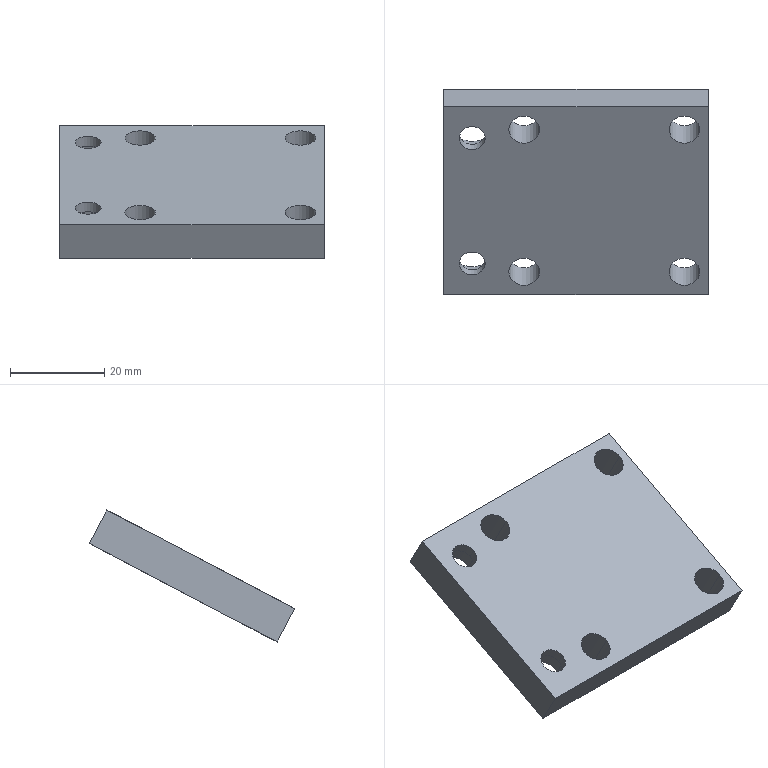Component | SolidWorks | SDACylinderFixingPlate-1 | 1 solid | 24 faces | box 56 x 43.56 x 28 mm | volume 18093 mm3 | cylinder 16 | plane 8 | commonest cylinder face diameters 6.5 x8 10 x4 5.5 x4
build123d program:
from build123d import *

# Parameters (mm, degrees)
SKETCH1_W                                          = 56
SKETCH1_H                                          = 45
BOSS_EXTRUDE1_DEPTH                                = 8
HOLE_SIZE_ACCORDING_TO_TYPE_1_OF_HEXAG_D           = 5.5
HOLE_SIZE_ACCORDING_TO_TYPE_1_OF_HEXAG_CBORE_D     = 10
HOLE_SIZE_ACCORDING_TO_TYPE_1_OF_HEXAG_CBORE_DEPTH = 5.7
F_6_5_6_5_DIAMETER_HOLE1_D                         = 6.5


with BuildPart() as part:
    # Sketch1 → Boss-Extrude1 (new body)
    with BuildSketch(Plane.XY):
        Rectangle(SKETCH1_W, SKETCH1_H)
    extrude(amount=BOSS_EXTRUDE1_DEPTH)

    # Hole Size _according to_ Type 1 of Hexag (through all)
    with Locations(Plane.XY.offset(8)):
        with Locations((22, 15), (22, -15)):
            CounterBoreHole(HOLE_SIZE_ACCORDING_TO_TYPE_1_OF_HEXAG_D / 2, HOLE_SIZE_ACCORDING_TO_TYPE_1_OF_HEXAG_CBORE_D / 2, HOLE_SIZE_ACCORDING_TO_TYPE_1_OF_HEXAG_CBORE_DEPTH)

    # 6.5 _6.5_ Diameter Hole1 (through all)
    with Locations(Plane.XY.offset(8)):
        with Locations((-23, 17), (11, 17), (11, -17), (-23, -17)):
            Hole(F_6_5_6_5_DIAMETER_HOLE1_D / 2)


solid = part.part

# Placed as in the assembly
solid = solid.moved(Location((-251.317, 16.632, 98.15), (-152.302, 0, 180)))
STEP:
#1=CARTESIAN_POINT('',(-8.861,1.247,4.175));
#2=VERTEX_POINT('',#1);
#3=CARTESIAN_POINT('',(-9.117,1.247,4.175));
#4=VERTEX_POINT('',#3);
#5=CARTESIAN_POINT('',(-8.989,1.247,4.175));
#6=DIRECTION('',(-0.,0.4648,-0.8854));
#7=DIRECTION('',(-1.,-0.,0.));
#8=AXIS2_PLACEMENT_3D('',#5,#6,#7);
#9=CIRCLE('',#8,0.128);
#10=EDGE_CURVE('',#2,#4,#9,.T.);
#11=ORIENTED_EDGE('',*,*,#10,.F.);
#12=CARTESIAN_POINT('',(-8.861,1.394,3.896));
#13=VERTEX_POINT('',#12);
#14=CARTESIAN_POINT('',(-8.861,1.394,3.896));
#15=DIRECTION('',(-0.,0.4648,-0.8854));
#16=VECTOR('',#15,39.37);
#17=LINE('',#14,#16);
#18=EDGE_CURVE('',#2,#13,#17,.T.);
#19=ORIENTED_EDGE('',*,*,#18,.T.);
#20=CARTESIAN_POINT('',(-9.117,1.394,3.896));
#21=VERTEX_POINT('',#20);
#22=CARTESIAN_POINT('',(-8.989,1.394,3.896));
#23=DIRECTION('',(-0.,0.4648,-0.8854));
#24=DIRECTION('',(-1.,-0.,0.));
#25=AXIS2_PLACEMENT_3D('',#22,#23,#24);
#26=CIRCLE('',#25,0.128);
#27=EDGE_CURVE('',#13,#21,#26,.T.);
#28=ORIENTED_EDGE('',*,*,#27,.T.);
#29=CARTESIAN_POINT('',(-9.117,1.394,3.896));
#30=DIRECTION('',(-0.,0.4648,-0.8854));
#31=VECTOR('',#30,39.37);
#32=LINE('',#29,#31);
#33=EDGE_CURVE('',#4,#21,#32,.T.);
#34=ORIENTED_EDGE('',*,*,#33,.F.);
#35=EDGE_LOOP('',(#11,#19,#28,#34));
#36=FACE_OUTER_BOUND('',#35,.T.);
#37=CARTESIAN_POINT('',(-8.989,1.394,3.896));
#38=DIRECTION('',(-0.,0.4648,-0.8854));
#39=DIRECTION('',(-1.,-0.,0.));
#40=AXIS2_PLACEMENT_3D('',#37,#38,#39);
#41=CYLINDRICAL_SURFACE('',#40,0.128);
#42=ADVANCED_FACE('',(#36),#41,.F.);
#43=CARTESIAN_POINT('',(-10.199,1.247,4.175));
#44=VERTEX_POINT('',#43);
#45=CARTESIAN_POINT('',(-10.455,1.247,4.175));
#46=VERTEX_POINT('',#45);
#47=CARTESIAN_POINT('',(-10.327,1.247,4.175));
#48=DIRECTION('',(-0.,0.4648,-0.8854));
#49=DIRECTION('',(-1.,-0.,0.));
#50=AXIS2_PLACEMENT_3D('',#47,#48,#49);
#51=CIRCLE('',#50,0.128);
#52=EDGE_CURVE('',#44,#46,#51,.T.);
#53=ORIENTED_EDGE('',*,*,#52,.F.);
#54=CARTESIAN_POINT('',(-10.199,1.394,3.896));
#55=VERTEX_POINT('',#54);
#56=CARTESIAN_POINT('',(-10.199,1.394,3.896));
#57=DIRECTION('',(-0.,0.4648,-0.8854));
#58=VECTOR('',#57,39.37);
#59=LINE('',#56,#58);
#60=EDGE_CURVE('',#44,#55,#59,.T.);
#61=ORIENTED_EDGE('',*,*,#60,.T.);
#62=CARTESIAN_POINT('',(-10.455,1.394,3.896));
#63=VERTEX_POINT('',#62);
#64=CARTESIAN_POINT('',(-10.327,1.394,3.896));
#65=DIRECTION('',(-0.,0.4648,-0.8854));
#66=DIRECTION('',(-1.,-0.,0.));
#67=AXIS2_PLACEMENT_3D('',#64,#65,#66);
#68=CIRCLE('',#67,0.128);
#69=EDGE_CURVE('',#55,#63,#68,.T.);
#70=ORIENTED_EDGE('',*,*,#69,.T.);
#71=CARTESIAN_POINT('',(-10.455,1.394,3.896));
#72=DIRECTION('',(-0.,0.4648,-0.8854));
#73=VECTOR('',#72,39.37);
#74=LINE('',#71,#73);
#75=EDGE_CURVE('',#46,#63,#74,.T.);
#76=ORIENTED_EDGE('',*,*,#75,.F.);
#77=EDGE_LOOP('',(#53,#61,#70,#76));
#78=FACE_OUTER_BOUND('',#77,.T.);
#79=CARTESIAN_POINT('',(-10.327,1.394,3.896));
#80=DIRECTION('',(-0.,0.4648,-0.8854));
#81=DIRECTION('',(-1.,-0.,0.));
#82=AXIS2_PLACEMENT_3D('',#79,#80,#81);
#83=CYLINDRICAL_SURFACE('',#82,0.128);
#84=ADVANCED_FACE('',(#78),#83,.F.);
#85=CARTESIAN_POINT('',(-10.199,0.06221,3.553));
#86=VERTEX_POINT('',#85);
#87=CARTESIAN_POINT('',(-10.455,0.06221,3.553));
#88=VERTEX_POINT('',#87);
#89=CARTESIAN_POINT('',(-10.327,0.06221,3.553));
#90=DIRECTION('',(-0.,0.4648,-0.8854));
#91=DIRECTION('',(-1.,-0.,0.));
#92=AXIS2_PLACEMENT_3D('',#89,#90,#91);
#93=CIRCLE('',#92,0.128);
#94=EDGE_CURVE('',#86,#88,#93,.T.);
#95=ORIENTED_EDGE('',*,*,#94,.F.);
#96=CARTESIAN_POINT('',(-10.199,0.2086,3.274));
#97=VERTEX_POINT('',#96);
#98=CARTESIAN_POINT('',(-10.199,0.2086,3.274));
#99=DIRECTION('',(-0.,0.4648,-0.8854));
#100=VECTOR('',#99,39.37);
#101=LINE('',#98,#100);
#102=EDGE_CURVE('',#86,#97,#101,.T.);
#103=ORIENTED_EDGE('',*,*,#102,.T.);
#104=CARTESIAN_POINT('',(-10.455,0.2086,3.274));
#105=VERTEX_POINT('',#104);
#106=CARTESIAN_POINT('',(-10.327,0.2086,3.274));
#107=DIRECTION('',(-0.,0.4648,-0.8854));
#108=DIRECTION('',(-1.,-0.,0.));
#109=AXIS2_PLACEMENT_3D('',#106,#107,#108);
#110=CIRCLE('',#109,0.128);
#111=EDGE_CURVE('',#97,#105,#110,.T.);
#112=ORIENTED_EDGE('',*,*,#111,.T.);
#113=CARTESIAN_POINT('',(-10.455,0.2086,3.274));
#114=DIRECTION('',(-0.,0.4648,-0.8854));
#115=VECTOR('',#114,39.37);
#116=LINE('',#113,#115);
#117=EDGE_CURVE('',#88,#105,#116,.T.);
#118=ORIENTED_EDGE('',*,*,#117,.F.);
#119=EDGE_LOOP('',(#95,#103,#112,#118));
#120=FACE_OUTER_BOUND('',#119,.T.);
#121=CARTESIAN_POINT('',(-10.327,0.2086,3.274));
#122=DIRECTION('',(-0.,0.4648,-0.8854));
#123=DIRECTION('',(-1.,-0.,0.));
#124=AXIS2_PLACEMENT_3D('',#121,#122,#123);
#125=CYLINDRICAL_SURFACE('',#124,0.128);
#126=ADVANCED_FACE('',(#120),#125,.F.);
#127=CARTESIAN_POINT('',(-8.861,0.06221,3.553));
#128=VERTEX_POINT('',#127);
#129=CARTESIAN_POINT('',(-9.117,0.06221,3.553));
#130=VERTEX_POINT('',#129);
#131=CARTESIAN_POINT('',(-8.989,0.06221,3.553));
#132=DIRECTION('',(-0.,0.4648,-0.8854));
#133=DIRECTION('',(-1.,-0.,0.));
#134=AXIS2_PLACEMENT_3D('',#131,#132,#133);
#135=CIRCLE('',#134,0.128);
#136=EDGE_CURVE('',#128,#130,#135,.T.);
#137=ORIENTED_EDGE('',*,*,#136,.F.);
#138=CARTESIAN_POINT('',(-8.861,0.2086,3.274));
#139=VERTEX_POINT('',#138);
#140=CARTESIAN_POINT('',(-8.861,0.2086,3.274));
#141=DIRECTION('',(-0.,0.4648,-0.8854));
#142=VECTOR('',#141,39.37);
#143=LINE('',#140,#142);
#144=EDGE_CURVE('',#128,#139,#143,.T.);
#145=ORIENTED_EDGE('',*,*,#144,.T.);
#146=CARTESIAN_POINT('',(-9.117,0.2086,3.274));
#147=VERTEX_POINT('',#146);
#148=CARTESIAN_POINT('',(-8.989,0.2086,3.274));
#149=DIRECTION('',(-0.,0.4648,-0.8854));
#150=DIRECTION('',(-1.,-0.,0.));
#151=AXIS2_PLACEMENT_3D('',#148,#149,#150);
#152=CIRCLE('',#151,0.128);
#153=EDGE_CURVE('',#139,#147,#152,.T.);
#154=ORIENTED_EDGE('',*,*,#153,.T.);
#155=CARTESIAN_POINT('',(-9.117,0.2086,3.274));
#156=DIRECTION('',(-0.,0.4648,-0.8854));
#157=VECTOR('',#156,39.37);
#158=LINE('',#155,#157);
#159=EDGE_CURVE('',#130,#147,#158,.T.);
#160=ORIENTED_EDGE('',*,*,#159,.F.);
#161=EDGE_LOOP('',(#137,#145,#154,#160));
#162=FACE_OUTER_BOUND('',#161,.T.);
#163=CARTESIAN_POINT('',(-8.989,0.2086,3.274));
#164=DIRECTION('',(-0.,0.4648,-0.8854));
#165=DIRECTION('',(-1.,-0.,0.));
#166=AXIS2_PLACEMENT_3D('',#163,#164,#165);
#167=CYLINDRICAL_SURFACE('',#166,0.128);
#168=ADVANCED_FACE('',(#162),#167,.F.);
#169=CARTESIAN_POINT('',(-10.564,1.22,4.058));
#170=VERTEX_POINT('',#169);
#171=CARTESIAN_POINT('',(-10.957,1.22,4.058));
#172=VERTEX_POINT('',#171);
#173=CARTESIAN_POINT('',(-10.76,1.22,4.058));
#174=DIRECTION('',(-0.,0.4648,-0.8854));
#175=DIRECTION('',(-1.,-0.,0.));
#176=AXIS2_PLACEMENT_3D('',#173,#174,#175);
#177=CIRCLE('',#176,0.1969);
#178=EDGE_CURVE('',#170,#172,#177,.T.);
#179=ORIENTED_EDGE('',*,*,#178,.F.);
#180=CARTESIAN_POINT('',(-10.564,1.324,3.86));
#181=VERTEX_POINT('',#180);
#182=CARTESIAN_POINT('',(-10.564,1.324,3.86));
#183=DIRECTION('',(-0.,0.4648,-0.8854));
#184=VECTOR('',#183,39.37);
#185=LINE('',#182,#184);
#186=EDGE_CURVE('',#170,#181,#185,.T.);
#187=ORIENTED_EDGE('',*,*,#186,.T.);
#188=CARTESIAN_POINT('',(-10.957,1.324,3.86));
#189=VERTEX_POINT('',#188);
#190=CARTESIAN_POINT('',(-10.76,1.324,3.86));
#191=DIRECTION('',(-0.,0.4648,-0.8854));
#192=DIRECTION('',(-1.,-0.,0.));
#193=AXIS2_PLACEMENT_3D('',#190,#191,#192);
#194=CIRCLE('',#193,0.1969);
#195=EDGE_CURVE('',#181,#189,#194,.T.);
#196=ORIENTED_EDGE('',*,*,#195,.T.);
#197=CARTESIAN_POINT('',(-10.957,1.324,3.86));
#198=DIRECTION('',(-0.,0.4648,-0.8854));
#199=VECTOR('',#198,39.37);
#200=LINE('',#197,#199);
#201=EDGE_CURVE('',#172,#189,#200,.T.);
#202=ORIENTED_EDGE('',*,*,#201,.F.);
#203=EDGE_LOOP('',(#179,#187,#196,#202));
#204=FACE_OUTER_BOUND('',#203,.T.);
#205=CARTESIAN_POINT('',(-10.76,1.324,3.86));
#206=DIRECTION('',(-0.,0.4648,-0.8854));
#207=DIRECTION('',(-1.,-0.,0.));
#208=AXIS2_PLACEMENT_3D('',#205,#206,#207);
#209=CYLINDRICAL_SURFACE('',#208,0.1969);
#210=ADVANCED_FACE('',(#204),#209,.F.);
#211=CARTESIAN_POINT('',(-10.652,1.178,4.139));
#212=VERTEX_POINT('',#211);
#213=CARTESIAN_POINT('',(-10.869,1.178,4.139));
#214=VERTEX_POINT('',#213);
#215=CARTESIAN_POINT('',(-10.76,1.178,4.139));
#216=DIRECTION('',(-0.,0.4648,-0.8854));
#217=DIRECTION('',(-1.,-0.,0.));
#218=AXIS2_PLACEMENT_3D('',#215,#216,#217);
#219=CIRCLE('',#218,0.1083);
#220=EDGE_CURVE('',#212,#214,#219,.T.);
#221=ORIENTED_EDGE('',*,*,#220,.F.);
#222=CARTESIAN_POINT('',(-10.652,1.22,4.058));
#223=VERTEX_POINT('',#222);
#224=CARTESIAN_POINT('',(-10.652,1.324,3.86));
#225=DIRECTION('',(-0.,0.4648,-0.8854));
#226=VECTOR('',#225,39.37);
#227=LINE('',#224,#226);
#228=EDGE_CURVE('',#212,#223,#227,.T.);
#229=ORIENTED_EDGE('',*,*,#228,.T.);
#230=CARTESIAN_POINT('',(-10.869,1.22,4.058));
#231=VERTEX_POINT('',#230);
#232=CARTESIAN_POINT('',(-10.76,1.22,4.058));
#233=DIRECTION('',(-0.,0.4648,-0.8854));
#234=DIRECTION('',(-1.,-0.,0.));
#235=AXIS2_PLACEMENT_3D('',#232,#233,#234);
#236=CIRCLE('',#235,0.1083);
#237=EDGE_CURVE('',#223,#231,#236,.T.);
#238=ORIENTED_EDGE('',*,*,#237,.T.);
#239=CARTESIAN_POINT('',(-10.869,1.324,3.86));
#240=DIRECTION('',(-0.,0.4648,-0.8854));
#241=VECTOR('',#240,39.37);
#242=LINE('',#239,#241);
#243=EDGE_CURVE('',#214,#231,#242,.T.);
#244=ORIENTED_EDGE('',*,*,#243,.F.);
#245=EDGE_LOOP('',(#221,#229,#238,#244));
#246=FACE_OUTER_BOUND('',#245,.T.);
#247=CARTESIAN_POINT('',(-10.76,1.324,3.86));
#248=DIRECTION('',(-0.,0.4648,-0.8854));
#249=DIRECTION('',(-1.,-0.,0.));
#250=AXIS2_PLACEMENT_3D('',#247,#248,#249);
#251=CYLINDRICAL_SURFACE('',#250,0.1083);
#252=ADVANCED_FACE('',(#246),#251,.F.);
#253=CARTESIAN_POINT('',(-10.564,0.174,3.509));
#254=VERTEX_POINT('',#253);
#255=CARTESIAN_POINT('',(-10.957,0.174,3.509));
#256=VERTEX_POINT('',#255);
#257=CARTESIAN_POINT('',(-10.76,0.174,3.509));
#258=DIRECTION('',(-0.,0.4648,-0.8854));
#259=DIRECTION('',(-1.,-0.,0.));
#260=AXIS2_PLACEMENT_3D('',#257,#258,#259);
#261=CIRCLE('',#260,0.1969);
#262=EDGE_CURVE('',#254,#256,#261,.T.);
#263=ORIENTED_EDGE('',*,*,#262,.F.);
#264=CARTESIAN_POINT('',(-10.564,0.2783,3.311));
#265=VERTEX_POINT('',#264);
#266=CARTESIAN_POINT('',(-10.564,0.2783,3.311));
#267=DIRECTION('',(-0.,0.4648,-0.8854));
#268=VECTOR('',#267,39.37);
#269=LINE('',#266,#268);
#270=EDGE_CURVE('',#254,#265,#269,.T.);
#271=ORIENTED_EDGE('',*,*,#270,.T.);
#272=CARTESIAN_POINT('',(-10.957,0.2783,3.311));
#273=VERTEX_POINT('',#272);
#274=CARTESIAN_POINT('',(-10.76,0.2783,3.311));
#275=DIRECTION('',(-0.,0.4648,-0.8854));
#276=DIRECTION('',(-1.,-0.,0.));
#277=AXIS2_PLACEMENT_3D('',#274,#275,#276);
#278=CIRCLE('',#277,0.1969);
#279=EDGE_CURVE('',#265,#273,#278,.T.);
#280=ORIENTED_EDGE('',*,*,#279,.T.);
#281=CARTESIAN_POINT('',(-10.957,0.2783,3.311));
#282=DIRECTION('',(-0.,0.4648,-0.8854));
#283=VECTOR('',#282,39.37);
#284=LINE('',#281,#283);
#285=EDGE_CURVE('',#256,#273,#284,.T.);
#286=ORIENTED_EDGE('',*,*,#285,.F.);
#287=EDGE_LOOP('',(#263,#271,#280,#286));
#288=FACE_OUTER_BOUND('',#287,.T.);
#289=CARTESIAN_POINT('',(-10.76,0.2783,3.311));
#290=DIRECTION('',(-0.,0.4648,-0.8854));
#291=DIRECTION('',(-1.,-0.,0.));
#292=AXIS2_PLACEMENT_3D('',#289,#290,#291);
#293=CYLINDRICAL_SURFACE('',#292,0.1969);
#294=ADVANCED_FACE('',(#288),#293,.F.);
#295=CARTESIAN_POINT('',(-10.652,0.1319,3.59));
#296=VERTEX_POINT('',#295);
#297=CARTESIAN_POINT('',(-10.869,0.1319,3.59));
#298=VERTEX_POINT('',#297);
#299=CARTESIAN_POINT('',(-10.76,0.1319,3.59));
#300=DIRECTION('',(-0.,0.4648,-0.8854));
#301=DIRECTION('',(-1.,-0.,0.));
#302=AXIS2_PLACEMENT_3D('',#299,#300,#301);
#303=CIRCLE('',#302,0.1083);
#304=EDGE_CURVE('',#296,#298,#303,.T.);
#305=ORIENTED_EDGE('',*,*,#304,.F.);
#306=CARTESIAN_POINT('',(-10.652,0.174,3.509));
#307=VERTEX_POINT('',#306);
#308=CARTESIAN_POINT('',(-10.652,0.2783,3.311));
#309=DIRECTION('',(-0.,0.4648,-0.8854));
#310=VECTOR('',#309,39.37);
#311=LINE('',#308,#310);
#312=EDGE_CURVE('',#296,#307,#311,.T.);
#313=ORIENTED_EDGE('',*,*,#312,.T.);
#314=CARTESIAN_POINT('',(-10.869,0.174,3.509));
#315=VERTEX_POINT('',#314);
#316=CARTESIAN_POINT('',(-10.76,0.174,3.509));
#317=DIRECTION('',(-0.,0.4648,-0.8854));
#318=DIRECTION('',(-1.,-0.,0.));
#319=AXIS2_PLACEMENT_3D('',#316,#317,#318);
#320=CIRCLE('',#319,0.1083);
#321=EDGE_CURVE('',#307,#315,#320,.T.);
#322=ORIENTED_EDGE('',*,*,#321,.T.);
#323=CARTESIAN_POINT('',(-10.869,0.2783,3.311));
#324=DIRECTION('',(-0.,0.4648,-0.8854));
#325=VECTOR('',#324,39.37);
#326=LINE('',#323,#325);
#327=EDGE_CURVE('',#298,#315,#326,.T.);
#328=ORIENTED_EDGE('',*,*,#327,.F.);
#329=EDGE_LOOP('',(#305,#313,#322,#328));
#330=FACE_OUTER_BOUND('',#329,.T.);
#331=CARTESIAN_POINT('',(-10.76,0.2783,3.311));
#332=DIRECTION('',(-0.,0.4648,-0.8854));
#333=DIRECTION('',(-1.,-0.,0.));
#334=AXIS2_PLACEMENT_3D('',#331,#332,#333);
#335=CYLINDRICAL_SURFACE('',#334,0.1083);
#336=ADVANCED_FACE('',(#330),#335,.F.);
#337=CARTESIAN_POINT('',(-10.997,-0.1295,3.452));
#338=VERTEX_POINT('',#337);
#339=CARTESIAN_POINT('',(-10.997,1.439,4.276));
#340=VERTEX_POINT('',#339);
#341=CARTESIAN_POINT('',(-10.997,-0.1295,3.452));
#342=DIRECTION('',(-0.,0.8854,0.4648));
#343=VECTOR('',#342,39.37);
#344=LINE('',#341,#343);
#345=EDGE_CURVE('',#338,#340,#344,.T.);
#346=ORIENTED_EDGE('',*,*,#345,.T.);
#347=CARTESIAN_POINT('',(-10.997,1.586,3.997));
#348=VERTEX_POINT('',#347);
#349=CARTESIAN_POINT('',(-10.997,1.586,3.997));
#350=DIRECTION('',(0.,-0.4648,0.8854));
#351=VECTOR('',#350,39.37);
#352=LINE('',#349,#351);
#353=EDGE_CURVE('',#348,#340,#352,.T.);
#354=ORIENTED_EDGE('',*,*,#353,.F.);
#355=CARTESIAN_POINT('',(-10.997,0.01689,3.174));
#356=VERTEX_POINT('',#355);
#357=CARTESIAN_POINT('',(-10.997,0.01689,3.174));
#358=DIRECTION('',(-0.,0.8854,0.4648));
#359=VECTOR('',#358,39.37);
#360=LINE('',#357,#359);
#361=EDGE_CURVE('',#356,#348,#360,.T.);
#362=ORIENTED_EDGE('',*,*,#361,.F.);
#363=CARTESIAN_POINT('',(-10.997,0.01689,3.174));
#364=DIRECTION('',(0.,-0.4648,0.8854));
#365=VECTOR('',#364,39.37);
#366=LINE('',#363,#365);
#367=EDGE_CURVE('',#356,#338,#366,.T.);
#368=ORIENTED_EDGE('',*,*,#367,.T.);
#369=EDGE_LOOP('',(#346,#354,#362,#368));
#370=FACE_OUTER_BOUND('',#369,.T.);
#371=CARTESIAN_POINT('',(-10.997,0.01689,3.174));
#372=DIRECTION('',(1.,0.,0.));
#373=DIRECTION('',(-0.,0.4648,-0.8854));
#374=AXIS2_PLACEMENT_3D('',#371,#372,#373);
#375=PLANE('',#374);
#376=ADVANCED_FACE('',(#370),#375,.F.);
#377=CARTESIAN_POINT('',(-8.792,1.439,4.276));
#378=VERTEX_POINT('',#377);
#379=CARTESIAN_POINT('',(-8.792,1.439,4.276));
#380=DIRECTION('',(1.,0.,0.));
#381=VECTOR('',#380,39.37);
#382=LINE('',#379,#381);
#383=EDGE_CURVE('',#340,#378,#382,.T.);
#384=ORIENTED_EDGE('',*,*,#383,.T.);
#385=CARTESIAN_POINT('',(-8.792,1.586,3.997));
#386=VERTEX_POINT('',#385);
#387=CARTESIAN_POINT('',(-8.792,1.586,3.997));
#388=DIRECTION('',(0.,-0.4648,0.8854));
#389=VECTOR('',#388,39.37);
#390=LINE('',#387,#389);
#391=EDGE_CURVE('',#386,#378,#390,.T.);
#392=ORIENTED_EDGE('',*,*,#391,.F.);
#393=CARTESIAN_POINT('',(-8.792,1.586,3.997));
#394=DIRECTION('',(1.,0.,0.));
#395=VECTOR('',#394,39.37);
#396=LINE('',#393,#395);
#397=EDGE_CURVE('',#348,#386,#396,.T.);
#398=ORIENTED_EDGE('',*,*,#397,.F.);
#399=ORIENTED_EDGE('',*,*,#353,.T.);
#400=EDGE_LOOP('',(#384,#392,#398,#399));
#401=FACE_OUTER_BOUND('',#400,.T.);
#402=CARTESIAN_POINT('',(-8.792,1.586,3.997));
#403=DIRECTION('',(0.,-0.8854,-0.4648));
#404=DIRECTION('',(0.,-0.4648,0.8854));
#405=AXIS2_PLACEMENT_3D('',#402,#403,#404);
#406=PLANE('',#405);
#407=ADVANCED_FACE('',(#401),#406,.F.);
#408=CARTESIAN_POINT('',(-8.792,-0.1295,3.452));
#409=VERTEX_POINT('',#408);
#410=CARTESIAN_POINT('',(-8.792,-0.1295,3.452));
#411=DIRECTION('',(0.,-0.8854,-0.4648));
#412=VECTOR('',#411,39.37);
#413=LINE('',#410,#412);
#414=EDGE_CURVE('',#378,#409,#413,.T.);
#415=ORIENTED_EDGE('',*,*,#414,.T.);
#416=CARTESIAN_POINT('',(-8.792,0.01689,3.174));
#417=VERTEX_POINT('',#416);
#418=CARTESIAN_POINT('',(-8.792,0.01689,3.174));
#419=DIRECTION('',(0.,-0.4648,0.8854));
#420=VECTOR('',#419,39.37);
#421=LINE('',#418,#420);
#422=EDGE_CURVE('',#417,#409,#421,.T.);
#423=ORIENTED_EDGE('',*,*,#422,.F.);
#424=CARTESIAN_POINT('',(-8.792,0.01689,3.174));
#425=DIRECTION('',(0.,-0.8854,-0.4648));
#426=VECTOR('',#425,39.37);
#427=LINE('',#424,#426);
#428=EDGE_CURVE('',#386,#417,#427,.T.);
#429=ORIENTED_EDGE('',*,*,#428,.F.);
#430=ORIENTED_EDGE('',*,*,#391,.T.);
#431=EDGE_LOOP('',(#415,#423,#429,#430));
#432=FACE_OUTER_BOUND('',#431,.T.);
#433=CARTESIAN_POINT('',(-8.792,0.01689,3.174));
#434=DIRECTION('',(-1.,-0.,-0.));
#435=DIRECTION('',(0.,-0.4648,0.8854));
#436=AXIS2_PLACEMENT_3D('',#433,#434,#435);
#437=PLANE('',#436);
#438=ADVANCED_FACE('',(#432),#437,.F.);
#439=CARTESIAN_POINT('',(-8.792,-0.1295,3.452));
#440=DIRECTION('',(-1.,-0.,-0.));
#441=VECTOR('',#440,39.37);
#442=LINE('',#439,#441);
#443=EDGE_CURVE('',#409,#338,#442,.T.);
#444=ORIENTED_EDGE('',*,*,#443,.T.);
#445=ORIENTED_EDGE('',*,*,#367,.F.);
#446=CARTESIAN_POINT('',(-8.792,0.01689,3.174));
#447=DIRECTION('',(-1.,-0.,-0.));
#448=VECTOR('',#447,39.37);
#449=LINE('',#446,#448);
#450=EDGE_CURVE('',#417,#356,#449,.T.);
#451=ORIENTED_EDGE('',*,*,#450,.F.);
#452=ORIENTED_EDGE('',*,*,#422,.T.);
#453=EDGE_LOOP('',(#444,#445,#451,#452));
#454=FACE_OUTER_BOUND('',#453,.T.);
#455=CARTESIAN_POINT('',(-8.792,0.01689,3.174));
#456=DIRECTION('',(-0.,0.8854,0.4648));
#457=DIRECTION('',(-0.,0.4648,-0.8854));
#458=AXIS2_PLACEMENT_3D('',#455,#456,#457);
#459=PLANE('',#458);
#460=ADVANCED_FACE('',(#454),#459,.F.);
#461=CARTESIAN_POINT('',(-8.989,1.394,3.896));
#462=DIRECTION('',(-0.,0.4648,-0.8854));
#463=DIRECTION('',(-1.,-0.,0.));
#464=AXIS2_PLACEMENT_3D('',#461,#462,#463);
#465=CIRCLE('',#464,0.128);
#466=EDGE_CURVE('',#21,#13,#465,.T.);
#467=ORIENTED_EDGE('',*,*,#466,.F.);
#468=ORIENTED_EDGE('',*,*,#27,.F.);
#469=EDGE_LOOP('',(#467,#468));
#470=FACE_BOUND('',#469,.T.);
#471=CARTESIAN_POINT('',(-10.327,1.394,3.896));
#472=DIRECTION('',(-0.,0.4648,-0.8854));
#473=DIRECTION('',(-1.,-0.,0.));
#474=AXIS2_PLACEMENT_3D('',#471,#472,#473);
#475=CIRCLE('',#474,0.128);
#476=EDGE_CURVE('',#63,#55,#475,.T.);
#477=ORIENTED_EDGE('',*,*,#476,.F.);
#478=ORIENTED_EDGE('',*,*,#69,.F.);
#479=EDGE_LOOP('',(#477,#478));
#480=FACE_BOUND('',#479,.T.);
#481=CARTESIAN_POINT('',(-10.327,0.2086,3.274));
#482=DIRECTION('',(-0.,0.4648,-0.8854));
#483=DIRECTION('',(-1.,-0.,0.));
#484=AXIS2_PLACEMENT_3D('',#481,#482,#483);
#485=CIRCLE('',#484,0.128);
#486=EDGE_CURVE('',#105,#97,#485,.T.);
#487=ORIENTED_EDGE('',*,*,#486,.F.);
#488=ORIENTED_EDGE('',*,*,#111,.F.);
#489=EDGE_LOOP('',(#487,#488));
#490=FACE_BOUND('',#489,.T.);
#491=CARTESIAN_POINT('',(-8.989,0.2086,3.274));
#492=DIRECTION('',(-0.,0.4648,-0.8854));
#493=DIRECTION('',(-1.,-0.,0.));
#494=AXIS2_PLACEMENT_3D('',#491,#492,#493);
#495=CIRCLE('',#494,0.128);
#496=EDGE_CURVE('',#147,#139,#495,.T.);
#497=ORIENTED_EDGE('',*,*,#496,.F.);
#498=ORIENTED_EDGE('',*,*,#153,.F.);
#499=EDGE_LOOP('',(#497,#498));
#500=FACE_BOUND('',#499,.T.);
#501=CARTESIAN_POINT('',(-10.76,1.324,3.86));
#502=DIRECTION('',(-0.,0.4648,-0.8854));
#503=DIRECTION('',(-1.,-0.,0.));
#504=AXIS2_PLACEMENT_3D('',#501,#502,#503);
#505=CIRCLE('',#504,0.1969);
#506=EDGE_CURVE('',#189,#181,#505,.T.);
#507=ORIENTED_EDGE('',*,*,#506,.F.);
#508=ORIENTED_EDGE('',*,*,#195,.F.);
#509=EDGE_LOOP('',(#507,#508));
#510=FACE_BOUND('',#509,.T.);
#511=CARTESIAN_POINT('',(-10.76,0.2783,3.311));
#512=DIRECTION('',(-0.,0.4648,-0.8854));
#513=DIRECTION('',(-1.,-0.,0.));
#514=AXIS2_PLACEMENT_3D('',#511,#512,#513);
#515=CIRCLE('',#514,0.1969);
#516=EDGE_CURVE('',#273,#265,#515,.T.);
#517=ORIENTED_EDGE('',*,*,#516,.F.);
#518=ORIENTED_EDGE('',*,*,#279,.F.);
#519=EDGE_LOOP('',(#517,#518));
#520=FACE_BOUND('',#519,.T.);
#521=ORIENTED_EDGE('',*,*,#361,.T.);
#522=ORIENTED_EDGE('',*,*,#397,.T.);
#523=ORIENTED_EDGE('',*,*,#428,.T.);
#524=ORIENTED_EDGE('',*,*,#450,.T.);
#525=EDGE_LOOP('',(#521,#522,#523,#524));
#526=FACE_OUTER_BOUND('',#525,.T.);
#527=CARTESIAN_POINT('',(-9.894,0.8012,3.585));
#528=DIRECTION('',(0.,-0.4648,0.8854));
#529=DIRECTION('',(1.,0.,0.));
#530=AXIS2_PLACEMENT_3D('',#527,#528,#529);
#531=PLANE('',#530);
#532=ADVANCED_FACE('',(#470,#480,#490,#500,#510,#520,#526),#531,.F.);
#533=CARTESIAN_POINT('',(-8.989,1.247,4.175));
#534=DIRECTION('',(-0.,0.4648,-0.8854));
#535=DIRECTION('',(-1.,-0.,0.));
#536=AXIS2_PLACEMENT_3D('',#533,#534,#535);
#537=CIRCLE('',#536,0.128);
#538=EDGE_CURVE('',#4,#2,#537,.T.);
#539=ORIENTED_EDGE('',*,*,#538,.T.);
#540=ORIENTED_EDGE('',*,*,#10,.T.);
#541=EDGE_LOOP('',(#539,#540));
#542=FACE_BOUND('',#541,.T.);
#543=CARTESIAN_POINT('',(-10.327,1.247,4.175));
#544=DIRECTION('',(-0.,0.4648,-0.8854));
#545=DIRECTION('',(-1.,-0.,0.));
#546=AXIS2_PLACEMENT_3D('',#543,#544,#545);
#547=CIRCLE('',#546,0.128);
#548=EDGE_CURVE('',#46,#44,#547,.T.);
#549=ORIENTED_EDGE('',*,*,#548,.T.);
#550=ORIENTED_EDGE('',*,*,#52,.T.);
#551=EDGE_LOOP('',(#549,#550));
#552=FACE_BOUND('',#551,.T.);
#553=CARTESIAN_POINT('',(-10.327,0.06221,3.553));
#554=DIRECTION('',(-0.,0.4648,-0.8854));
#555=DIRECTION('',(-1.,-0.,0.));
#556=AXIS2_PLACEMENT_3D('',#553,#554,#555);
#557=CIRCLE('',#556,0.128);
#558=EDGE_CURVE('',#88,#86,#557,.T.);
#559=ORIENTED_EDGE('',*,*,#558,.T.);
#560=ORIENTED_EDGE('',*,*,#94,.T.);
#561=EDGE_LOOP('',(#559,#560));
#562=FACE_BOUND('',#561,.T.);
#563=CARTESIAN_POINT('',(-8.989,0.06221,3.553));
#564=DIRECTION('',(-0.,0.4648,-0.8854));
#565=DIRECTION('',(-1.,-0.,0.));
#566=AXIS2_PLACEMENT_3D('',#563,#564,#565);
#567=CIRCLE('',#566,0.128);
#568=EDGE_CURVE('',#130,#128,#567,.T.);
#569=ORIENTED_EDGE('',*,*,#568,.T.);
#570=ORIENTED_EDGE('',*,*,#136,.T.);
#571=EDGE_LOOP('',(#569,#570));
#572=FACE_BOUND('',#571,.T.);
#573=CARTESIAN_POINT('',(-10.76,1.178,4.139));
#574=DIRECTION('',(-0.,0.4648,-0.8854));
#575=DIRECTION('',(-1.,-0.,0.));
#576=AXIS2_PLACEMENT_3D('',#573,#574,#575);
#577=CIRCLE('',#576,0.1083);
#578=EDGE_CURVE('',#214,#212,#577,.T.);
#579=ORIENTED_EDGE('',*,*,#578,.T.);
#580=ORIENTED_EDGE('',*,*,#220,.T.);
#581=EDGE_LOOP('',(#579,#580));
#582=FACE_BOUND('',#581,.T.);
#583=CARTESIAN_POINT('',(-10.76,0.1319,3.59));
#584=DIRECTION('',(-0.,0.4648,-0.8854));
#585=DIRECTION('',(-1.,-0.,0.));
#586=AXIS2_PLACEMENT_3D('',#583,#584,#585);
#587=CIRCLE('',#586,0.1083);
#588=EDGE_CURVE('',#298,#296,#587,.T.);
#589=ORIENTED_EDGE('',*,*,#588,.T.);
#590=ORIENTED_EDGE('',*,*,#304,.T.);
#591=EDGE_LOOP('',(#589,#590));
#592=FACE_BOUND('',#591,.T.);
#593=ORIENTED_EDGE('',*,*,#345,.F.);
#594=ORIENTED_EDGE('',*,*,#443,.F.);
#595=ORIENTED_EDGE('',*,*,#414,.F.);
#596=ORIENTED_EDGE('',*,*,#383,.F.);
#597=EDGE_LOOP('',(#593,#594,#595,#596));
#598=FACE_OUTER_BOUND('',#597,.T.);
#599=CARTESIAN_POINT('',(-9.894,0.6548,3.864));
#600=DIRECTION('',(0.,-0.4648,0.8854));
#601=DIRECTION('',(1.,0.,0.));
#602=AXIS2_PLACEMENT_3D('',#599,#600,#601);
#603=PLANE('',#602);
#604=ADVANCED_FACE('',(#542,#552,#562,#572,#582,#592,#598),#603,.T.);
#605=ORIENTED_EDGE('',*,*,#312,.F.);
#606=ORIENTED_EDGE('',*,*,#588,.F.);
#607=ORIENTED_EDGE('',*,*,#327,.T.);
#608=CARTESIAN_POINT('',(-10.76,0.174,3.509));
#609=DIRECTION('',(-0.,0.4648,-0.8854));
#610=DIRECTION('',(-1.,-0.,0.));
#611=AXIS2_PLACEMENT_3D('',#608,#609,#610);
#612=CIRCLE('',#611,0.1083);
#613=EDGE_CURVE('',#315,#307,#612,.T.);
#614=ORIENTED_EDGE('',*,*,#613,.T.);
#615=EDGE_LOOP('',(#605,#606,#607,#614));
#616=FACE_OUTER_BOUND('',#615,.T.);
#617=CARTESIAN_POINT('',(-10.76,0.2783,3.311));
#618=DIRECTION('',(-0.,0.4648,-0.8854));
#619=DIRECTION('',(-1.,-0.,0.));
#620=AXIS2_PLACEMENT_3D('',#617,#618,#619);
#621=CYLINDRICAL_SURFACE('',#620,0.1083);
#622=ADVANCED_FACE('',(#616),#621,.F.);
#623=ORIENTED_EDGE('',*,*,#613,.F.);
#624=ORIENTED_EDGE('',*,*,#321,.F.);
#625=EDGE_LOOP('',(#623,#624));
#626=FACE_BOUND('',#625,.T.);
#627=CARTESIAN_POINT('',(-10.76,0.174,3.509));
#628=DIRECTION('',(-0.,0.4648,-0.8854));
#629=DIRECTION('',(-1.,-0.,0.));
#630=AXIS2_PLACEMENT_3D('',#627,#628,#629);
#631=CIRCLE('',#630,0.1969);
#632=EDGE_CURVE('',#256,#254,#631,.T.);
#633=ORIENTED_EDGE('',*,*,#632,.T.);
#634=ORIENTED_EDGE('',*,*,#262,.T.);
#635=EDGE_LOOP('',(#633,#634));
#636=FACE_OUTER_BOUND('',#635,.T.);
#637=CARTESIAN_POINT('',(-10.869,0.174,3.509));
#638=DIRECTION('',(0.,-0.4648,0.8854));
#639=DIRECTION('',(1.,0.,0.));
#640=AXIS2_PLACEMENT_3D('',#637,#638,#639);
#641=PLANE('',#640);
#642=ADVANCED_FACE('',(#626,#636),#641,.F.);
#643=ORIENTED_EDGE('',*,*,#270,.F.);
#644=ORIENTED_EDGE('',*,*,#632,.F.);
#645=ORIENTED_EDGE('',*,*,#285,.T.);
#646=ORIENTED_EDGE('',*,*,#516,.T.);
#647=EDGE_LOOP('',(#643,#644,#645,#646));
#648=FACE_OUTER_BOUND('',#647,.T.);
#649=CARTESIAN_POINT('',(-10.76,0.2783,3.311));
#650=DIRECTION('',(-0.,0.4648,-0.8854));
#651=DIRECTION('',(-1.,-0.,0.));
#652=AXIS2_PLACEMENT_3D('',#649,#650,#651);
#653=CYLINDRICAL_SURFACE('',#652,0.1969);
#654=ADVANCED_FACE('',(#648),#653,.F.);
#655=ORIENTED_EDGE('',*,*,#228,.F.);
#656=ORIENTED_EDGE('',*,*,#578,.F.);
#657=ORIENTED_EDGE('',*,*,#243,.T.);
#658=CARTESIAN_POINT('',(-10.76,1.22,4.058));
#659=DIRECTION('',(-0.,0.4648,-0.8854));
#660=DIRECTION('',(-1.,-0.,0.));
#661=AXIS2_PLACEMENT_3D('',#658,#659,#660);
#662=CIRCLE('',#661,0.1083);
#663=EDGE_CURVE('',#231,#223,#662,.T.);
#664=ORIENTED_EDGE('',*,*,#663,.T.);
#665=EDGE_LOOP('',(#655,#656,#657,#664));
#666=FACE_OUTER_BOUND('',#665,.T.);
#667=CARTESIAN_POINT('',(-10.76,1.324,3.86));
#668=DIRECTION('',(-0.,0.4648,-0.8854));
#669=DIRECTION('',(-1.,-0.,0.));
#670=AXIS2_PLACEMENT_3D('',#667,#668,#669);
#671=CYLINDRICAL_SURFACE('',#670,0.1083);
#672=ADVANCED_FACE('',(#666),#671,.F.);
#673=ORIENTED_EDGE('',*,*,#663,.F.);
#674=ORIENTED_EDGE('',*,*,#237,.F.);
#675=EDGE_LOOP('',(#673,#674));
#676=FACE_BOUND('',#675,.T.);
#677=CARTESIAN_POINT('',(-10.76,1.22,4.058));
#678=DIRECTION('',(-0.,0.4648,-0.8854));
#679=DIRECTION('',(-1.,-0.,0.));
#680=AXIS2_PLACEMENT_3D('',#677,#678,#679);
#681=CIRCLE('',#680,0.1969);
#682=EDGE_CURVE('',#172,#170,#681,.T.);
#683=ORIENTED_EDGE('',*,*,#682,.T.);
#684=ORIENTED_EDGE('',*,*,#178,.T.);
#685=EDGE_LOOP('',(#683,#684));
#686=FACE_OUTER_BOUND('',#685,.T.);
#687=CARTESIAN_POINT('',(-10.869,1.22,4.058));
#688=DIRECTION('',(0.,-0.4648,0.8854));
#689=DIRECTION('',(1.,0.,0.));
#690=AXIS2_PLACEMENT_3D('',#687,#688,#689);
#691=PLANE('',#690);
#692=ADVANCED_FACE('',(#676,#686),#691,.F.);
#693=ORIENTED_EDGE('',*,*,#186,.F.);
#694=ORIENTED_EDGE('',*,*,#682,.F.);
#695=ORIENTED_EDGE('',*,*,#201,.T.);
#696=ORIENTED_EDGE('',*,*,#506,.T.);
#697=EDGE_LOOP('',(#693,#694,#695,#696));
#698=FACE_OUTER_BOUND('',#697,.T.);
#699=CARTESIAN_POINT('',(-10.76,1.324,3.86));
#700=DIRECTION('',(-0.,0.4648,-0.8854));
#701=DIRECTION('',(-1.,-0.,0.));
#702=AXIS2_PLACEMENT_3D('',#699,#700,#701);
#703=CYLINDRICAL_SURFACE('',#702,0.1969);
#704=ADVANCED_FACE('',(#698),#703,.F.);
#705=ORIENTED_EDGE('',*,*,#144,.F.);
#706=ORIENTED_EDGE('',*,*,#568,.F.);
#707=ORIENTED_EDGE('',*,*,#159,.T.);
#708=ORIENTED_EDGE('',*,*,#496,.T.);
#709=EDGE_LOOP('',(#705,#706,#707,#708));
#710=FACE_OUTER_BOUND('',#709,.T.);
#711=CARTESIAN_POINT('',(-8.989,0.2086,3.274));
#712=DIRECTION('',(-0.,0.4648,-0.8854));
#713=DIRECTION('',(-1.,-0.,0.));
#714=AXIS2_PLACEMENT_3D('',#711,#712,#713);
#715=CYLINDRICAL_SURFACE('',#714,0.128);
#716=ADVANCED_FACE('',(#710),#715,.F.);
#717=ORIENTED_EDGE('',*,*,#102,.F.);
#718=ORIENTED_EDGE('',*,*,#558,.F.);
#719=ORIENTED_EDGE('',*,*,#117,.T.);
#720=ORIENTED_EDGE('',*,*,#486,.T.);
#721=EDGE_LOOP('',(#717,#718,#719,#720));
#722=FACE_OUTER_BOUND('',#721,.T.);
#723=CARTESIAN_POINT('',(-10.327,0.2086,3.274));
#724=DIRECTION('',(-0.,0.4648,-0.8854));
#725=DIRECTION('',(-1.,-0.,0.));
#726=AXIS2_PLACEMENT_3D('',#723,#724,#725);
#727=CYLINDRICAL_SURFACE('',#726,0.128);
#728=ADVANCED_FACE('',(#722),#727,.F.);
#729=ORIENTED_EDGE('',*,*,#60,.F.);
#730=ORIENTED_EDGE('',*,*,#548,.F.);
#731=ORIENTED_EDGE('',*,*,#75,.T.);
#732=ORIENTED_EDGE('',*,*,#476,.T.);
#733=EDGE_LOOP('',(#729,#730,#731,#732));
#734=FACE_OUTER_BOUND('',#733,.T.);
#735=CARTESIAN_POINT('',(-10.327,1.394,3.896));
#736=DIRECTION('',(-0.,0.4648,-0.8854));
#737=DIRECTION('',(-1.,-0.,0.));
#738=AXIS2_PLACEMENT_3D('',#735,#736,#737);
#739=CYLINDRICAL_SURFACE('',#738,0.128);
#740=ADVANCED_FACE('',(#734),#739,.F.);
#741=ORIENTED_EDGE('',*,*,#18,.F.);
#742=ORIENTED_EDGE('',*,*,#538,.F.);
#743=ORIENTED_EDGE('',*,*,#33,.T.);
#744=ORIENTED_EDGE('',*,*,#466,.T.);
#745=EDGE_LOOP('',(#741,#742,#743,#744));
#746=FACE_OUTER_BOUND('',#745,.T.);
#747=CARTESIAN_POINT('',(-8.989,1.394,3.896));
#748=DIRECTION('',(-0.,0.4648,-0.8854));
#749=DIRECTION('',(-1.,-0.,0.));
#750=AXIS2_PLACEMENT_3D('',#747,#748,#749);
#751=CYLINDRICAL_SURFACE('',#750,0.128);
#752=ADVANCED_FACE('',(#746),#751,.F.);
#753=CLOSED_SHELL('',(#42,#84,#126,#168,#210,#252,#294,#336,#376,#407,#438,#460,#532,#604,#622,#642,#654,#672,#692,#704,#716,#728,#740,#752));
#754=MANIFOLD_SOLID_BREP('',#753);
#755=CARTESIAN_POINT('',(0.,0.,0.));
#756=DIRECTION('',(0.,0.,1.));
#757=DIRECTION('',(1.,0.,0.));
#758=AXIS2_PLACEMENT_3D('',#755,#756,#757);
#759=(LENGTH_UNIT()NAMED_UNIT(*)SI_UNIT($,.METRE.));
#760=LENGTH_MEASURE_WITH_UNIT(LENGTH_MEASURE(0.0254),#759);
#761=DIMENSIONAL_EXPONENTS(1.,0.,0.,0.,0.,0.,0.);
#762=(CONVERSION_BASED_UNIT('',#760)LENGTH_UNIT()NAMED_UNIT(#761));
#763=UNCERTAINTY_MEASURE_WITH_UNIT(LENGTH_MEASURE(0.00001),#762,'','');
#764=(NAMED_UNIT(*)PLANE_ANGLE_UNIT()SI_UNIT($,.RADIAN.));
#765=(NAMED_UNIT(*)SI_UNIT($,.STERADIAN.)SOLID_ANGLE_UNIT());
#766=(GEOMETRIC_REPRESENTATION_CONTEXT(3)GLOBAL_UNCERTAINTY_ASSIGNED_CONTEXT((#763))GLOBAL_UNIT_ASSIGNED_CONTEXT((#762,#764,#765))REPRESENTATION_CONTEXT('',''));
#767=ADVANCED_BREP_SHAPE_REPRESENTATION('',(#754,#758),#766);
#768=COLOUR_RGB('',0.7922,0.8196,0.9333);
#769=FILL_AREA_STYLE_COLOUR('',#768);
#770=FILL_AREA_STYLE('',(#769));
#771=SURFACE_STYLE_FILL_AREA(#770);
#772=SURFACE_SIDE_STYLE('',(#771));
#773=SURFACE_STYLE_USAGE(.BOTH.,#772);
#774=PRESENTATION_STYLE_ASSIGNMENT((#773));
#775=STYLED_ITEM('',(#774),#754);
#776=PRESENTATION_LAYER_ASSIGNMENT('','',(#775));
#777=(LENGTH_UNIT()NAMED_UNIT(*)SI_UNIT($,.METRE.));
#778=LENGTH_MEASURE_WITH_UNIT(LENGTH_MEASURE(0.0254),#777);
#779=DIMENSIONAL_EXPONENTS(1.,0.,0.,0.,0.,0.,0.);
#780=(CONVERSION_BASED_UNIT('',#778)LENGTH_UNIT()NAMED_UNIT(#779));
#781=UNCERTAINTY_MEASURE_WITH_UNIT(LENGTH_MEASURE(0.00001),#780,'','');
#782=(NAMED_UNIT(*)PLANE_ANGLE_UNIT()SI_UNIT($,.RADIAN.));
#783=(NAMED_UNIT(*)SI_UNIT($,.STERADIAN.)SOLID_ANGLE_UNIT());
#784=(GEOMETRIC_REPRESENTATION_CONTEXT(3)GLOBAL_UNCERTAINTY_ASSIGNED_CONTEXT((#781))GLOBAL_UNIT_ASSIGNED_CONTEXT((#780,#782,#783))REPRESENTATION_CONTEXT('',''));
#785=MECHANICAL_DESIGN_GEOMETRIC_PRESENTATION_REPRESENTATION('',(#775),#784);